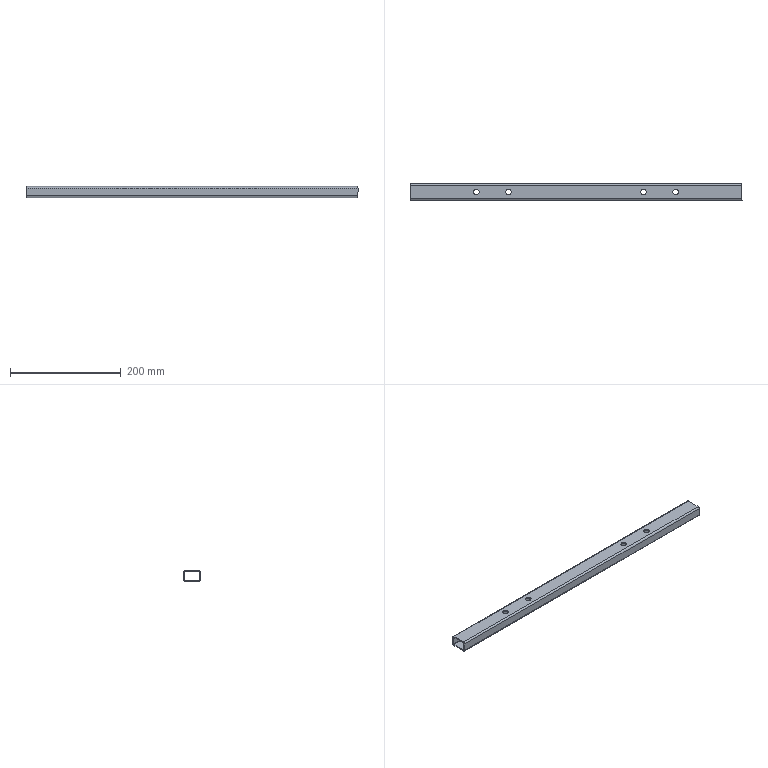Component | SolidWorks | CleaningRobotAssembly-1_30x20x2RectangularColdBentHollowSectionSteel900MM-2 | 1 solid | 34 faces | box 600 x 30 x 20 mm | volume 105023 mm3 | cylinder 24 | plane 10 | commonest cylinder face diameters 10 x16 6 x4 2 x4
build123d program:
from build123d import *

# Parameters (mm, degrees)
BOSS_EXTRUDE1_DEPTH = 600
SKETCH7_R           = 5
CUT_EXTRUDE1_DEPTH  = 83


with BuildPart() as part:
    # Sketch1 → Boss-Extrude1 (new body)
    with BuildSketch(Plane(origin=(0, 0, 0), x_dir=(0, 0, -1), z_dir=(1, 0, 0))):
        with BuildLine():
            Line((-6.263, 13), (6.263, 13))
            Line((6.263, 13), (7.561, 14.947))
            ThreePointArc((7.561, 14.947), (7.282, 14.987), (7, 15))
            Line((7, 15), (-7, 15))
            ThreePointArc((-7, 15), (-7.282, 14.987), (-7.561, 14.947))
            Line((-7.561, 14.947), (-6.263, 13))
        make_face()
        with BuildLine():
            Line((-10, -11.394), (-8, -8.394))
            Line((-8, -8.394), (-8, 12))
            ThreePointArc((-8, 12), (-7.707, 12.707), (-7, 13))
            Line((-7, 13), (-6.263, 13))
            Line((-6.263, 13), (-7.561, 14.947))
            ThreePointArc((-7.561, 14.947), (-9.311, 13.913), (-10, 12))
            Line((-10, 12), (-10, -11.394))
        make_face()
        with BuildLine():
            Line((8, 12), (8, -8.394))
            Line((8, -8.394), (10, -11.394))
            Line((10, -11.394), (10, 12))
            ThreePointArc((10, 12), (9.311, 13.913), (7.561, 14.947))
            Line((7.561, 14.947), (6.263, 13))
            Line((6.263, 13), (7, 13))
            ThreePointArc((7, 13), (7.707, 12.707), (8, 12))
        make_face()
        with BuildLine():
            Line((7, -13), (-7, -13))
            ThreePointArc((-7, -13), (-7.707, -12.707), (-8, -12))
            Line((-8, -12), (-8, -8.394))
            Line((-8, -8.394), (-10, -11.394))
            Line((-10, -11.394), (-10, -12))
            ThreePointArc((-10, -12), (-9.121, -14.121), (-7, -15))
            Line((-7, -15), (7, -15))
            ThreePointArc((7, -15), (9.121, -14.121), (10, -12))
            Line((10, -12), (10, -11.394))
            Line((10, -11.394), (8, -8.394))
            Line((8, -8.394), (8, -12))
            ThreePointArc((8, -12), (7.707, -12.707), (7, -13))
        make_face()
    extrude(amount=BOSS_EXTRUDE1_DEPTH)

    # Sketch7 → Cut-Extrude1 (cut)
    with BuildSketch(Plane.XY.offset(10)):
        with Locations((120, 0)):
            Circle(SKETCH7_R)
        with Locations((178, 0)):
            Circle(SKETCH7_R)
    cut_extrude1 = extrude(amount=-CUT_EXTRUDE1_DEPTH, mode=Mode.SUBTRACT)

    # Mirror2: Cut-Extrude1 across plane
    add(cut_extrude1.mirror(Plane.ZY.offset(-300)), mode=Mode.SUBTRACT)


solid = part.part

# Placed as in the assembly
solid = solid.moved(Location((-274.371, -272.9, 228), (0, 0, 0)))